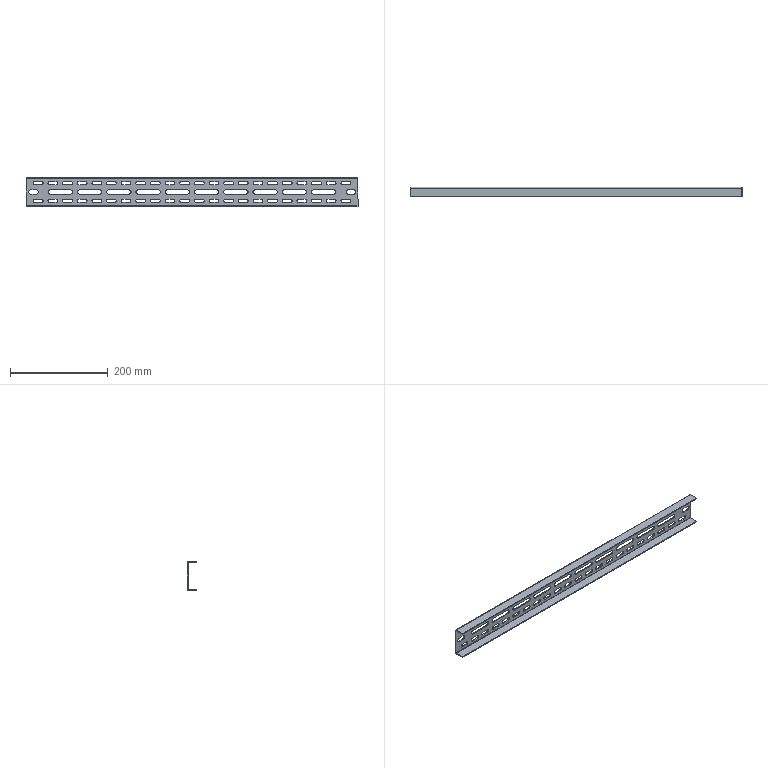Component | SolidWorks | MountingBeam-1 | 1 solid | 302 faces | volume 108111 mm3 | cylinder 172 | plane 130 | commonest cylinder face diameters 7 x132 9 x36 5 x2 1 x2